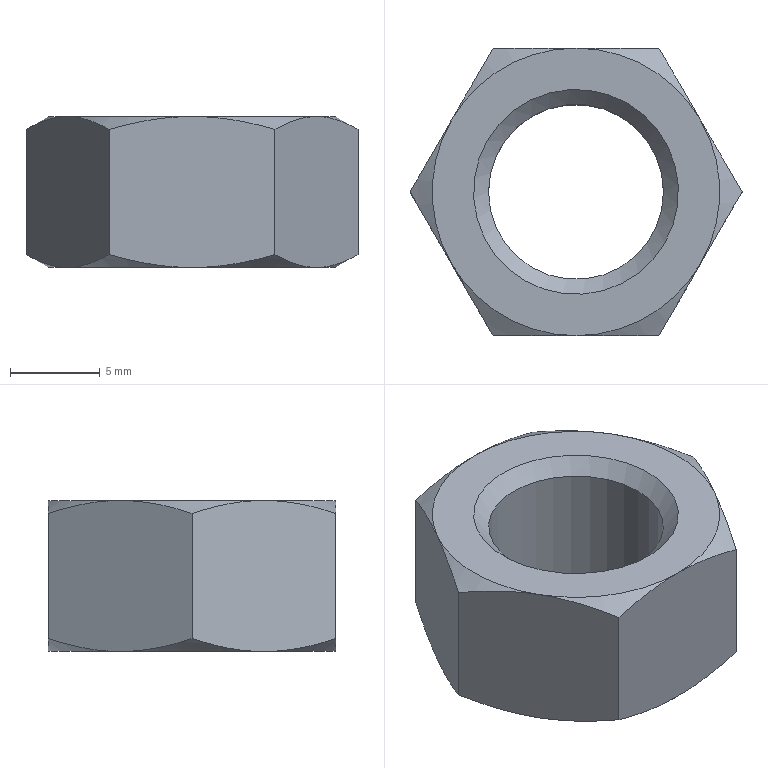Component | NX | GB-T6170_F-2000_M10X1_5_11 | 1 solid | 23 faces | volume 1206 mm3 | cone 14 | plane 8 | cylinder 1 | commonest cylinder face diameters 9.732 x1